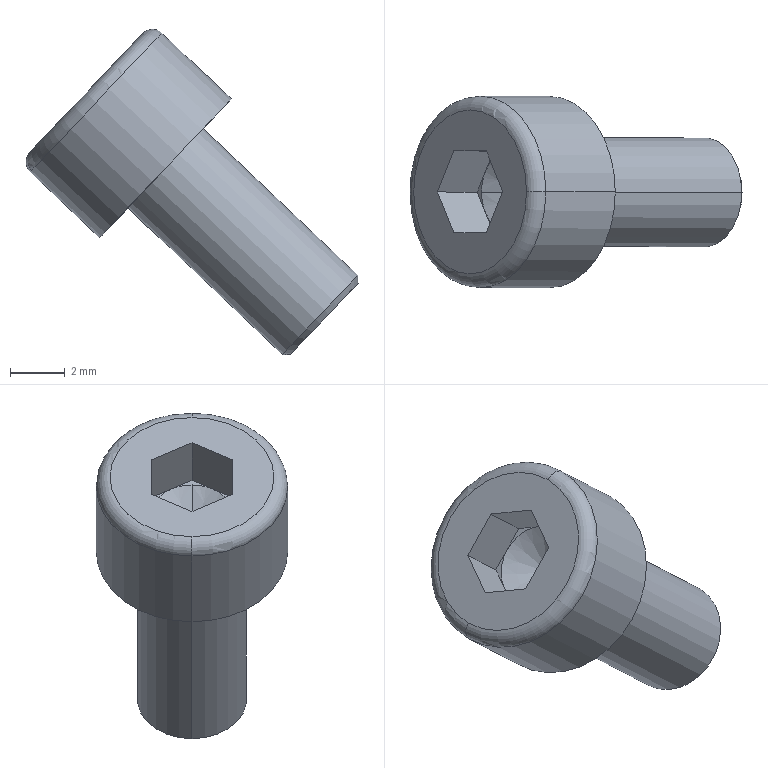Component | SolidWorks | 100-1_hexagon socket head cap screws gb_GB_FASTENER_SCREWS_HSHCS M4X8-N-1 | 1 solid | 25 faces | box 12.15 x 7 x 11.9 mm | volume 235 mm3 | plane 15 | cone 4 | cylinder 4 | torus 2 | commonest cylinder face diameters 4 x2 7 x2
STEP:
#1=COLOUR_RGB('',0.7922,0.8196,0.9333);
#2=FILL_AREA_STYLE_COLOUR('',#1);
#3=FILL_AREA_STYLE('',(#2));
#4=SURFACE_STYLE_FILL_AREA(#3);
#5=SURFACE_SIDE_STYLE('',(#4));
#6=SURFACE_STYLE_USAGE(.BOTH.,#5);
#7=PRESENTATION_STYLE_ASSIGNMENT((#6));
#8=CARTESIAN_POINT('',(20.34,50.315,-80.234));
#9=VERTEX_POINT('',#8);
#10=CARTESIAN_POINT('',(20.34,50.315,-80.222));
#11=VERTEX_POINT('',#10);
#12=CARTESIAN_POINT('',(20.34,50.315,-80.234));
#13=DIRECTION('',(-0.02683,-0.,0.9996));
#14=VECTOR('',#13,39.37);
#15=LINE('',#12,#14);
#16=EDGE_CURVE('',#9,#11,#15,.T.);
#17=ORIENTED_EDGE('',*,*,#16,.F.);
#18=CARTESIAN_POINT('',(20.242,50.315,-80.336));
#19=VERTEX_POINT('',#18);
#20=CARTESIAN_POINT('',(20.291,50.315,-80.285));
#21=DIRECTION('',(0.7258,0.,-0.6879));
#22=DIRECTION('',(0.6879,-0.,0.7258));
#23=AXIS2_PLACEMENT_3D('',#20,#21,#22);
#24=CIRCLE('',#23,0.07087);
#25=EDGE_CURVE('',#19,#9,#24,.T.);
#26=ORIENTED_EDGE('',*,*,#25,.F.);
#27=CARTESIAN_POINT('',(20.231,50.315,-80.337));
#28=VERTEX_POINT('',#27);
#29=CARTESIAN_POINT('',(20.242,50.315,-80.336));
#30=DIRECTION('',(-0.9996,0.,-0.02683));
#31=VECTOR('',#30,39.37);
#32=LINE('',#29,#31);
#33=EDGE_CURVE('',#19,#28,#32,.T.);
#34=ORIENTED_EDGE('',*,*,#33,.T.);
#35=CARTESIAN_POINT('',(20.285,50.315,-80.28));
#36=DIRECTION('',(-0.7258,-0.,0.6879));
#37=DIRECTION('',(0.6879,-0.,0.7258));
#38=AXIS2_PLACEMENT_3D('',#35,#36,#37);
#39=CIRCLE('',#38,0.07874);
#40=EDGE_CURVE('',#11,#28,#39,.T.);
#41=ORIENTED_EDGE('',*,*,#40,.F.);
#42=EDGE_LOOP('',(#17,#26,#34,#41));
#43=FACE_OUTER_BOUND('',#42,.T.);
#44=CARTESIAN_POINT('',(20.291,50.315,-80.285));
#45=DIRECTION('',(-0.7258,-0.,0.6879));
#46=DIRECTION('',(-0.6879,0.,-0.7258));
#47=AXIS2_PLACEMENT_3D('',#44,#45,#46);
#48=CONICAL_SURFACE('',#47,0.07087,0.7854);
#49=ADVANCED_FACE('',(#43),#48,.T.);
#50=CARTESIAN_POINT('',(19.867,50.315,-80.046));
#51=VERTEX_POINT('',#50);
#52=CARTESIAN_POINT('',(19.868,50.315,-80.074));
#53=VERTEX_POINT('',#52);
#54=CARTESIAN_POINT('',(19.881,50.315,-80.059));
#55=DIRECTION('',(-0.,-1.,-0.));
#56=DIRECTION('',(-0.6879,0.,-0.7258));
#57=AXIS2_PLACEMENT_3D('',#54,#55,#56);
#58=CIRCLE('',#57,0.01969);
#59=EDGE_CURVE('',#51,#53,#58,.T.);
#60=ORIENTED_EDGE('',*,*,#59,.F.);
#61=CARTESIAN_POINT('',(20.029,50.315,-79.874));
#62=VERTEX_POINT('',#61);
#63=CARTESIAN_POINT('',(19.948,50.315,-79.96));
#64=DIRECTION('',(-0.7258,-0.,0.6879));
#65=DIRECTION('',(0.6879,-0.,0.7258));
#66=AXIS2_PLACEMENT_3D('',#63,#64,#65);
#67=CIRCLE('',#66,0.1181);
#68=EDGE_CURVE('',#62,#51,#67,.T.);
#69=ORIENTED_EDGE('',*,*,#68,.F.);
#70=CARTESIAN_POINT('',(20.057,50.315,-79.874));
#71=VERTEX_POINT('',#70);
#72=CARTESIAN_POINT('',(20.044,50.315,-79.888));
#73=DIRECTION('',(0.,1.,0.));
#74=DIRECTION('',(0.6879,0.,0.7258));
#75=AXIS2_PLACEMENT_3D('',#72,#73,#74);
#76=CIRCLE('',#75,0.01969);
#77=EDGE_CURVE('',#62,#71,#76,.T.);
#78=ORIENTED_EDGE('',*,*,#77,.T.);
#79=CARTESIAN_POINT('',(19.963,50.315,-79.974));
#80=DIRECTION('',(0.7258,0.,-0.6879));
#81=DIRECTION('',(0.6879,-0.,0.7258));
#82=AXIS2_PLACEMENT_3D('',#79,#80,#81);
#83=CIRCLE('',#82,0.1378);
#84=EDGE_CURVE('',#53,#71,#83,.T.);
#85=ORIENTED_EDGE('',*,*,#84,.F.);
#86=EDGE_LOOP('',(#60,#69,#78,#85));
#87=FACE_OUTER_BOUND('',#86,.T.);
#88=CARTESIAN_POINT('',(19.963,50.315,-79.974));
#89=DIRECTION('',(0.7258,0.,-0.6879));
#90=DIRECTION('',(0.6879,-0.,0.7258));
#91=AXIS2_PLACEMENT_3D('',#88,#89,#90);
#92=TOROIDAL_SURFACE('',#91,0.1181,0.01969);
#93=ADVANCED_FACE('',(#87),#92,.T.);
#94=CARTESIAN_POINT('',(20.03,50.315,-80.038));
#95=VERTEX_POINT('',#94);
#96=CARTESIAN_POINT('',(20.046,50.315,-79.971));
#97=VERTEX_POINT('',#96);
#98=CARTESIAN_POINT('',(20.046,50.315,-79.971));
#99=DIRECTION('',(0.2328,-0.,0.9725));
#100=VECTOR('',#99,39.37);
#101=LINE('',#98,#100);
#102=EDGE_CURVE('',#95,#97,#101,.T.);
#103=ORIENTED_EDGE('',*,*,#102,.F.);
#104=CARTESIAN_POINT('',(19.965,50.315,-80.057));
#105=VERTEX_POINT('',#104);
#106=CARTESIAN_POINT('',(19.965,50.315,-80.057));
#107=DIRECTION('',(-0.9586,0.,-0.2846));
#108=VECTOR('',#107,39.37);
#109=LINE('',#106,#108);
#110=EDGE_CURVE('',#95,#105,#109,.T.);
#111=ORIENTED_EDGE('',*,*,#110,.T.);
#112=CARTESIAN_POINT('',(19.97,50.285,-80.051));
#113=VERTEX_POINT('',#112);
#114=CARTESIAN_POINT('',(20.005,50.315,-80.014));
#115=DIRECTION('',(-0.7258,-0.,0.6879));
#116=DIRECTION('',(0.6879,-0.,0.7258));
#117=AXIS2_PLACEMENT_3D('',#114,#115,#116);
#118=CIRCLE('',#117,0.05906);
#119=EDGE_CURVE('',#105,#113,#118,.T.);
#120=ORIENTED_EDGE('',*,*,#119,.T.);
#121=CARTESIAN_POINT('',(20.005,50.256,-80.014));
#122=VERTEX_POINT('',#121);
#123=CARTESIAN_POINT('',(20.005,50.315,-80.014));
#124=DIRECTION('',(-0.7258,-0.,0.6879));
#125=DIRECTION('',(0.6879,-0.,0.7258));
#126=AXIS2_PLACEMENT_3D('',#123,#124,#125);
#127=CIRCLE('',#126,0.05906);
#128=EDGE_CURVE('',#113,#122,#127,.T.);
#129=ORIENTED_EDGE('',*,*,#128,.T.);
#130=CARTESIAN_POINT('',(20.041,50.285,-79.977));
#131=VERTEX_POINT('',#130);
#132=CARTESIAN_POINT('',(20.005,50.315,-80.014));
#133=DIRECTION('',(0.7258,0.,-0.6879));
#134=DIRECTION('',(0.6879,-0.,0.7258));
#135=AXIS2_PLACEMENT_3D('',#132,#133,#134);
#136=CIRCLE('',#135,0.05906);
#137=EDGE_CURVE('',#131,#122,#136,.T.);
#138=ORIENTED_EDGE('',*,*,#137,.F.);
#139=CARTESIAN_POINT('',(20.005,50.315,-80.014));
#140=DIRECTION('',(-0.7258,-0.,0.6879));
#141=DIRECTION('',(0.6879,-0.,0.7258));
#142=AXIS2_PLACEMENT_3D('',#139,#140,#141);
#143=CIRCLE('',#142,0.05906);
#144=EDGE_CURVE('',#131,#97,#143,.T.);
#145=ORIENTED_EDGE('',*,*,#144,.T.);
#146=EDGE_LOOP('',(#103,#111,#120,#129,#138,#145));
#147=FACE_OUTER_BOUND('',#146,.T.);
#148=CARTESIAN_POINT('',(20.005,50.315,-80.014));
#149=DIRECTION('',(-0.7258,-0.,0.6879));
#150=DIRECTION('',(-0.6879,0.,-0.7258));
#151=AXIS2_PLACEMENT_3D('',#148,#149,#150);
#152=CONICAL_SURFACE('',#151,0.05906,1.047);
#153=ADVANCED_FACE('',(#147),#152,.F.);
#154=CARTESIAN_POINT('',(19.925,50.374,-79.985));
#155=VERTEX_POINT('',#154);
#156=CARTESIAN_POINT('',(19.972,50.374,-79.935));
#157=VERTEX_POINT('',#156);
#158=CARTESIAN_POINT('',(19.925,50.374,-79.985));
#159=DIRECTION('',(0.6879,-0.,0.7258));
#160=VECTOR('',#159,39.37);
#161=LINE('',#158,#160);
#162=EDGE_CURVE('',#155,#157,#161,.T.);
#163=ORIENTED_EDGE('',*,*,#162,.F.);
#164=CARTESIAN_POINT('',(19.982,50.374,-80.039));
#165=VERTEX_POINT('',#164);
#166=CARTESIAN_POINT('',(19.982,50.374,-80.039));
#167=DIRECTION('',(-0.7258,-0.,0.6879));
#168=VECTOR('',#167,39.37);
#169=LINE('',#166,#168);
#170=EDGE_CURVE('',#165,#155,#169,.T.);
#171=ORIENTED_EDGE('',*,*,#170,.F.);
#172=CARTESIAN_POINT('',(20.005,50.374,-80.014));
#173=VERTEX_POINT('',#172);
#174=CARTESIAN_POINT('',(19.982,50.374,-80.039));
#175=DIRECTION('',(0.6879,-0.,0.7258));
#176=VECTOR('',#175,39.37);
#177=LINE('',#174,#176);
#178=EDGE_CURVE('',#165,#173,#177,.T.);
#179=ORIENTED_EDGE('',*,*,#178,.T.);
#180=CARTESIAN_POINT('',(20.029,50.374,-79.989));
#181=VERTEX_POINT('',#180);
#182=CARTESIAN_POINT('',(19.982,50.374,-80.039));
#183=DIRECTION('',(0.6879,-0.,0.7258));
#184=VECTOR('',#183,39.37);
#185=LINE('',#182,#184);
#186=EDGE_CURVE('',#173,#181,#185,.T.);
#187=ORIENTED_EDGE('',*,*,#186,.T.);
#188=CARTESIAN_POINT('',(20.029,50.374,-79.989));
#189=DIRECTION('',(-0.7258,-0.,0.6879));
#190=VECTOR('',#189,39.37);
#191=LINE('',#188,#190);
#192=EDGE_CURVE('',#181,#157,#191,.T.);
#193=ORIENTED_EDGE('',*,*,#192,.T.);
#194=EDGE_LOOP('',(#163,#171,#179,#187,#193));
#195=FACE_OUTER_BOUND('',#194,.T.);
#196=CARTESIAN_POINT('',(19.982,50.374,-80.039));
#197=DIRECTION('',(-0.,-1.,-0.));
#198=DIRECTION('',(0.6879,-0.,0.7258));
#199=AXIS2_PLACEMENT_3D('',#196,#197,#198);
#200=PLANE('',#199);
#201=ADVANCED_FACE('',(#195),#200,.T.);
#202=CARTESIAN_POINT('',(19.901,50.315,-80.01));
#203=VERTEX_POINT('',#202);
#204=CARTESIAN_POINT('',(19.901,50.315,-80.01));
#205=DIRECTION('',(0.3439,0.866,0.3629));
#206=VECTOR('',#205,39.37);
#207=LINE('',#204,#206);
#208=EDGE_CURVE('',#203,#155,#207,.T.);
#209=ORIENTED_EDGE('',*,*,#208,.F.);
#210=CARTESIAN_POINT('',(19.958,50.315,-80.064));
#211=VERTEX_POINT('',#210);
#212=CARTESIAN_POINT('',(19.958,50.315,-80.064));
#213=DIRECTION('',(-0.7258,-0.,0.6879));
#214=VECTOR('',#213,39.37);
#215=LINE('',#212,#214);
#216=EDGE_CURVE('',#211,#203,#215,.T.);
#217=ORIENTED_EDGE('',*,*,#216,.F.);
#218=CARTESIAN_POINT('',(19.97,50.344,-80.051));
#219=VERTEX_POINT('',#218);
#220=CARTESIAN_POINT('',(19.958,50.315,-80.064));
#221=DIRECTION('',(0.3439,0.866,0.3629));
#222=VECTOR('',#221,39.37);
#223=LINE('',#220,#222);
#224=EDGE_CURVE('',#211,#219,#223,.T.);
#225=ORIENTED_EDGE('',*,*,#224,.T.);
#226=CARTESIAN_POINT('',(19.958,50.315,-80.064));
#227=DIRECTION('',(0.3439,0.866,0.3629));
#228=VECTOR('',#227,39.37);
#229=LINE('',#226,#228);
#230=EDGE_CURVE('',#219,#165,#229,.T.);
#231=ORIENTED_EDGE('',*,*,#230,.T.);
#232=ORIENTED_EDGE('',*,*,#170,.T.);
#233=EDGE_LOOP('',(#209,#217,#225,#231,#232));
#234=FACE_OUTER_BOUND('',#233,.T.);
#235=CARTESIAN_POINT('',(19.958,50.315,-80.064));
#236=DIRECTION('',(0.5957,-0.5,0.6286));
#237=DIRECTION('',(-0.7258,-0.,0.6879));
#238=AXIS2_PLACEMENT_3D('',#235,#236,#237);
#239=PLANE('',#238);
#240=ADVANCED_FACE('',(#234),#239,.T.);
#241=CARTESIAN_POINT('',(19.925,50.256,-79.985));
#242=VERTEX_POINT('',#241);
#243=CARTESIAN_POINT('',(19.925,50.256,-79.985));
#244=DIRECTION('',(-0.3439,0.866,-0.3629));
#245=VECTOR('',#244,39.37);
#246=LINE('',#243,#245);
#247=EDGE_CURVE('',#242,#203,#246,.T.);
#248=ORIENTED_EDGE('',*,*,#247,.F.);
#249=CARTESIAN_POINT('',(19.982,50.256,-80.039));
#250=VERTEX_POINT('',#249);
#251=CARTESIAN_POINT('',(19.982,50.256,-80.039));
#252=DIRECTION('',(-0.7258,-0.,0.6879));
#253=VECTOR('',#252,39.37);
#254=LINE('',#251,#253);
#255=EDGE_CURVE('',#250,#242,#254,.T.);
#256=ORIENTED_EDGE('',*,*,#255,.F.);
#257=CARTESIAN_POINT('',(19.982,50.256,-80.039));
#258=DIRECTION('',(-0.3439,0.866,-0.3629));
#259=VECTOR('',#258,39.37);
#260=LINE('',#257,#259);
#261=EDGE_CURVE('',#250,#113,#260,.T.);
#262=ORIENTED_EDGE('',*,*,#261,.T.);
#263=CARTESIAN_POINT('',(19.982,50.256,-80.039));
#264=DIRECTION('',(-0.3439,0.866,-0.3629));
#265=VECTOR('',#264,39.37);
#266=LINE('',#263,#265);
#267=EDGE_CURVE('',#113,#211,#266,.T.);
#268=ORIENTED_EDGE('',*,*,#267,.T.);
#269=ORIENTED_EDGE('',*,*,#216,.T.);
#270=EDGE_LOOP('',(#248,#256,#262,#268,#269));
#271=FACE_OUTER_BOUND('',#270,.T.);
#272=CARTESIAN_POINT('',(19.982,50.256,-80.039));
#273=DIRECTION('',(0.5957,0.5,0.6286));
#274=DIRECTION('',(-0.3439,0.866,-0.3629));
#275=AXIS2_PLACEMENT_3D('',#272,#273,#274);
#276=PLANE('',#275);
#277=ADVANCED_FACE('',(#271),#276,.T.);
#278=CARTESIAN_POINT('',(19.972,50.256,-79.935));
#279=VERTEX_POINT('',#278);
#280=CARTESIAN_POINT('',(19.972,50.256,-79.935));
#281=DIRECTION('',(-0.6879,0.,-0.7258));
#282=VECTOR('',#281,39.37);
#283=LINE('',#280,#282);
#284=EDGE_CURVE('',#279,#242,#283,.T.);
#285=ORIENTED_EDGE('',*,*,#284,.F.);
#286=CARTESIAN_POINT('',(20.029,50.256,-79.989));
#287=VERTEX_POINT('',#286);
#288=CARTESIAN_POINT('',(20.029,50.256,-79.989));
#289=DIRECTION('',(-0.7258,-0.,0.6879));
#290=VECTOR('',#289,39.37);
#291=LINE('',#288,#290);
#292=EDGE_CURVE('',#287,#279,#291,.T.);
#293=ORIENTED_EDGE('',*,*,#292,.F.);
#294=CARTESIAN_POINT('',(20.029,50.256,-79.989));
#295=DIRECTION('',(-0.6879,0.,-0.7258));
#296=VECTOR('',#295,39.37);
#297=LINE('',#294,#296);
#298=EDGE_CURVE('',#287,#122,#297,.T.);
#299=ORIENTED_EDGE('',*,*,#298,.T.);
#300=CARTESIAN_POINT('',(20.029,50.256,-79.989));
#301=DIRECTION('',(-0.6879,0.,-0.7258));
#302=VECTOR('',#301,39.37);
#303=LINE('',#300,#302);
#304=EDGE_CURVE('',#122,#250,#303,.T.);
#305=ORIENTED_EDGE('',*,*,#304,.T.);
#306=ORIENTED_EDGE('',*,*,#255,.T.);
#307=EDGE_LOOP('',(#285,#293,#299,#305,#306));
#308=FACE_OUTER_BOUND('',#307,.T.);
#309=CARTESIAN_POINT('',(20.029,50.256,-79.989));
#310=DIRECTION('',(0.,1.,0.));
#311=DIRECTION('',(0.6879,-0.,0.7258));
#312=AXIS2_PLACEMENT_3D('',#309,#310,#311);
#313=PLANE('',#312);
#314=ADVANCED_FACE('',(#308),#313,.T.);
#315=CARTESIAN_POINT('',(19.995,50.315,-79.911));
#316=VERTEX_POINT('',#315);
#317=CARTESIAN_POINT('',(19.995,50.315,-79.911));
#318=DIRECTION('',(-0.3439,-0.866,-0.3629));
#319=VECTOR('',#318,39.37);
#320=LINE('',#317,#319);
#321=EDGE_CURVE('',#316,#279,#320,.T.);
#322=ORIENTED_EDGE('',*,*,#321,.F.);
#323=CARTESIAN_POINT('',(20.052,50.315,-79.965));
#324=VERTEX_POINT('',#323);
#325=CARTESIAN_POINT('',(20.052,50.315,-79.965));
#326=DIRECTION('',(-0.7258,-0.,0.6879));
#327=VECTOR('',#326,39.37);
#328=LINE('',#325,#327);
#329=EDGE_CURVE('',#324,#316,#328,.T.);
#330=ORIENTED_EDGE('',*,*,#329,.F.);
#331=CARTESIAN_POINT('',(20.052,50.315,-79.965));
#332=DIRECTION('',(-0.3439,-0.866,-0.3629));
#333=VECTOR('',#332,39.37);
#334=LINE('',#331,#333);
#335=EDGE_CURVE('',#324,#131,#334,.T.);
#336=ORIENTED_EDGE('',*,*,#335,.T.);
#337=CARTESIAN_POINT('',(20.052,50.315,-79.965));
#338=DIRECTION('',(-0.3439,-0.866,-0.3629));
#339=VECTOR('',#338,39.37);
#340=LINE('',#337,#339);
#341=EDGE_CURVE('',#131,#287,#340,.T.);
#342=ORIENTED_EDGE('',*,*,#341,.T.);
#343=ORIENTED_EDGE('',*,*,#292,.T.);
#344=EDGE_LOOP('',(#322,#330,#336,#342,#343));
#345=FACE_OUTER_BOUND('',#344,.T.);
#346=CARTESIAN_POINT('',(20.052,50.315,-79.965));
#347=DIRECTION('',(-0.5957,0.5,-0.6286));
#348=DIRECTION('',(-0.7258,-0.,0.6879));
#349=AXIS2_PLACEMENT_3D('',#346,#347,#348);
#350=PLANE('',#349);
#351=ADVANCED_FACE('',(#345),#350,.T.);
#352=CARTESIAN_POINT('',(19.972,50.374,-79.935));
#353=DIRECTION('',(0.3439,-0.866,0.3629));
#354=VECTOR('',#353,39.37);
#355=LINE('',#352,#354);
#356=EDGE_CURVE('',#157,#316,#355,.T.);
#357=ORIENTED_EDGE('',*,*,#356,.F.);
#358=ORIENTED_EDGE('',*,*,#192,.F.);
#359=CARTESIAN_POINT('',(20.041,50.344,-79.977));
#360=VERTEX_POINT('',#359);
#361=CARTESIAN_POINT('',(20.029,50.374,-79.989));
#362=DIRECTION('',(0.3439,-0.866,0.3629));
#363=VECTOR('',#362,39.37);
#364=LINE('',#361,#363);
#365=EDGE_CURVE('',#181,#360,#364,.T.);
#366=ORIENTED_EDGE('',*,*,#365,.T.);
#367=CARTESIAN_POINT('',(20.029,50.374,-79.989));
#368=DIRECTION('',(0.3439,-0.866,0.3629));
#369=VECTOR('',#368,39.37);
#370=LINE('',#367,#369);
#371=EDGE_CURVE('',#360,#324,#370,.T.);
#372=ORIENTED_EDGE('',*,*,#371,.T.);
#373=ORIENTED_EDGE('',*,*,#329,.T.);
#374=EDGE_LOOP('',(#357,#358,#366,#372,#373));
#375=FACE_OUTER_BOUND('',#374,.T.);
#376=CARTESIAN_POINT('',(20.029,50.374,-79.989));
#377=DIRECTION('',(-0.5957,-0.5,-0.6286));
#378=DIRECTION('',(0.7258,0.,-0.6879));
#379=AXIS2_PLACEMENT_3D('',#376,#377,#378);
#380=PLANE('',#379);
#381=ADVANCED_FACE('',(#375),#380,.T.);
#382=ORIENTED_EDGE('',*,*,#25,.T.);
#383=CARTESIAN_POINT('',(20.291,50.315,-80.285));
#384=DIRECTION('',(0.7258,0.,-0.6879));
#385=DIRECTION('',(0.6879,-0.,0.7258));
#386=AXIS2_PLACEMENT_3D('',#383,#384,#385);
#387=CIRCLE('',#386,0.07087);
#388=EDGE_CURVE('',#9,#19,#387,.T.);
#389=ORIENTED_EDGE('',*,*,#388,.T.);
#390=EDGE_LOOP('',(#382,#389));
#391=FACE_OUTER_BOUND('',#390,.T.);
#392=CARTESIAN_POINT('',(20.291,50.315,-80.285));
#393=DIRECTION('',(0.7258,0.,-0.6879));
#394=DIRECTION('',(-0.,-1.,-0.));
#395=AXIS2_PLACEMENT_3D('',#392,#393,#394);
#396=PLANE('',#395);
#397=ADVANCED_FACE('',(#391),#396,.T.);
#398=CARTESIAN_POINT('',(20.117,50.315,-80.011));
#399=VERTEX_POINT('',#398);
#400=CARTESIAN_POINT('',(20.345,50.315,-80.228));
#401=DIRECTION('',(-0.7258,-0.,0.6879));
#402=VECTOR('',#401,39.37);
#403=LINE('',#400,#402);
#404=EDGE_CURVE('',#11,#399,#403,.T.);
#405=ORIENTED_EDGE('',*,*,#404,.F.);
#406=ORIENTED_EDGE('',*,*,#40,.T.);
#407=CARTESIAN_POINT('',(20.008,50.315,-80.126));
#408=VERTEX_POINT('',#407);
#409=CARTESIAN_POINT('',(20.237,50.315,-80.342));
#410=DIRECTION('',(-0.7258,-0.,0.6879));
#411=VECTOR('',#410,39.37);
#412=LINE('',#409,#411);
#413=EDGE_CURVE('',#28,#408,#412,.T.);
#414=ORIENTED_EDGE('',*,*,#413,.T.);
#415=CARTESIAN_POINT('',(20.063,50.315,-80.068));
#416=DIRECTION('',(0.7258,0.,-0.6879));
#417=DIRECTION('',(0.6879,-0.,0.7258));
#418=AXIS2_PLACEMENT_3D('',#415,#416,#417);
#419=CIRCLE('',#418,0.07874);
#420=EDGE_CURVE('',#408,#399,#419,.T.);
#421=ORIENTED_EDGE('',*,*,#420,.T.);
#422=EDGE_LOOP('',(#405,#406,#414,#421));
#423=FACE_OUTER_BOUND('',#422,.T.);
#424=CARTESIAN_POINT('',(20.291,50.315,-80.285));
#425=DIRECTION('',(-0.7258,-0.,0.6879));
#426=DIRECTION('',(-0.6879,0.,-0.7258));
#427=AXIS2_PLACEMENT_3D('',#424,#425,#426);
#428=CYLINDRICAL_SURFACE('',#427,0.07874);
#429=ADVANCED_FACE('',(#423),#428,.T.);
#430=CARTESIAN_POINT('',(20.157,50.315,-79.968));
#431=VERTEX_POINT('',#430);
#432=CARTESIAN_POINT('',(20.157,50.315,-79.968));
#433=DIRECTION('',(-0.7258,-0.,0.6879));
#434=VECTOR('',#433,39.37);
#435=LINE('',#432,#434);
#436=EDGE_CURVE('',#431,#71,#435,.T.);
#437=ORIENTED_EDGE('',*,*,#436,.F.);
#438=CARTESIAN_POINT('',(19.968,50.315,-80.168));
#439=VERTEX_POINT('',#438);
#440=CARTESIAN_POINT('',(20.063,50.315,-80.068));
#441=DIRECTION('',(0.7258,0.,-0.6879));
#442=DIRECTION('',(0.6879,-0.,0.7258));
#443=AXIS2_PLACEMENT_3D('',#440,#441,#442);
#444=CIRCLE('',#443,0.1378);
#445=EDGE_CURVE('',#439,#431,#444,.T.);
#446=ORIENTED_EDGE('',*,*,#445,.F.);
#447=CARTESIAN_POINT('',(19.968,50.315,-80.168));
#448=DIRECTION('',(-0.7258,-0.,0.6879));
#449=VECTOR('',#448,39.37);
#450=LINE('',#447,#449);
#451=EDGE_CURVE('',#439,#53,#450,.T.);
#452=ORIENTED_EDGE('',*,*,#451,.T.);
#453=ORIENTED_EDGE('',*,*,#84,.T.);
#454=EDGE_LOOP('',(#437,#446,#452,#453));
#455=FACE_OUTER_BOUND('',#454,.T.);
#456=CARTESIAN_POINT('',(20.063,50.315,-80.068));
#457=DIRECTION('',(-0.7258,-0.,0.6879));
#458=DIRECTION('',(-0.6879,0.,-0.7258));
#459=AXIS2_PLACEMENT_3D('',#456,#457,#458);
#460=CYLINDRICAL_SURFACE('',#459,0.1378);
#461=ADVANCED_FACE('',(#455),#460,.T.);
#462=ORIENTED_EDGE('',*,*,#420,.F.);
#463=CARTESIAN_POINT('',(20.063,50.315,-80.068));
#464=DIRECTION('',(0.7258,0.,-0.6879));
#465=DIRECTION('',(0.6879,-0.,0.7258));
#466=AXIS2_PLACEMENT_3D('',#463,#464,#465);
#467=CIRCLE('',#466,0.07874);
#468=EDGE_CURVE('',#399,#408,#467,.T.);
#469=ORIENTED_EDGE('',*,*,#468,.F.);
#470=EDGE_LOOP('',(#462,#469));
#471=FACE_BOUND('',#470,.T.);
#472=ORIENTED_EDGE('',*,*,#445,.T.);
#473=CARTESIAN_POINT('',(20.063,50.315,-80.068));
#474=DIRECTION('',(0.7258,0.,-0.6879));
#475=DIRECTION('',(0.6879,-0.,0.7258));
#476=AXIS2_PLACEMENT_3D('',#473,#474,#475);
#477=CIRCLE('',#476,0.1378);
#478=EDGE_CURVE('',#431,#439,#477,.T.);
#479=ORIENTED_EDGE('',*,*,#478,.T.);
#480=EDGE_LOOP('',(#472,#479));
#481=FACE_OUTER_BOUND('',#480,.T.);
#482=CARTESIAN_POINT('',(20.063,50.315,-80.068));
#483=DIRECTION('',(0.7258,0.,-0.6879));
#484=DIRECTION('',(-0.,-1.,-0.));
#485=AXIS2_PLACEMENT_3D('',#482,#483,#484);
#486=PLANE('',#485);
#487=ADVANCED_FACE('',(#471,#481),#486,.T.);
#488=ORIENTED_EDGE('',*,*,#356,.T.);
#489=ORIENTED_EDGE('',*,*,#321,.T.);
#490=ORIENTED_EDGE('',*,*,#284,.T.);
#491=ORIENTED_EDGE('',*,*,#247,.T.);
#492=ORIENTED_EDGE('',*,*,#208,.T.);
#493=ORIENTED_EDGE('',*,*,#162,.T.);
#494=EDGE_LOOP('',(#488,#489,#490,#491,#492,#493));
#495=FACE_BOUND('',#494,.T.);
#496=ORIENTED_EDGE('',*,*,#68,.T.);
#497=CARTESIAN_POINT('',(19.948,50.315,-79.96));
#498=DIRECTION('',(-0.7258,-0.,0.6879));
#499=DIRECTION('',(0.6879,-0.,0.7258));
#500=AXIS2_PLACEMENT_3D('',#497,#498,#499);
#501=CIRCLE('',#500,0.1181);
#502=EDGE_CURVE('',#51,#62,#501,.T.);
#503=ORIENTED_EDGE('',*,*,#502,.T.);
#504=EDGE_LOOP('',(#496,#503));
#505=FACE_OUTER_BOUND('',#504,.T.);
#506=CARTESIAN_POINT('',(19.948,50.315,-79.96));
#507=DIRECTION('',(0.7258,0.,-0.6879));
#508=DIRECTION('',(-0.,-1.,-0.));
#509=AXIS2_PLACEMENT_3D('',#506,#507,#508);
#510=PLANE('',#509);
#511=ADVANCED_FACE('',(#495,#505),#510,.F.);
#512=ORIENTED_EDGE('',*,*,#144,.F.);
#513=ORIENTED_EDGE('',*,*,#335,.F.);
#514=ORIENTED_EDGE('',*,*,#371,.F.);
#515=CARTESIAN_POINT('',(20.005,50.315,-80.014));
#516=DIRECTION('',(-0.7258,-0.,0.6879));
#517=DIRECTION('',(0.6879,-0.,0.7258));
#518=AXIS2_PLACEMENT_3D('',#515,#516,#517);
#519=CIRCLE('',#518,0.05906);
#520=EDGE_CURVE('',#97,#360,#519,.T.);
#521=ORIENTED_EDGE('',*,*,#520,.F.);
#522=EDGE_LOOP('',(#512,#513,#514,#521));
#523=FACE_OUTER_BOUND('',#522,.T.);
#524=CARTESIAN_POINT('',(20.052,50.315,-79.965));
#525=DIRECTION('',(0.7258,0.,-0.6879));
#526=DIRECTION('',(-0.,-1.,-0.));
#527=AXIS2_PLACEMENT_3D('',#524,#525,#526);
#528=PLANE('',#527);
#529=ADVANCED_FACE('',(#523),#528,.F.);
#530=ORIENTED_EDGE('',*,*,#137,.T.);
#531=ORIENTED_EDGE('',*,*,#298,.F.);
#532=ORIENTED_EDGE('',*,*,#341,.F.);
#533=EDGE_LOOP('',(#530,#531,#532));
#534=FACE_OUTER_BOUND('',#533,.T.);
#535=CARTESIAN_POINT('',(20.052,50.315,-79.965));
#536=DIRECTION('',(0.7258,0.,-0.6879));
#537=DIRECTION('',(-0.,-1.,-0.));
#538=AXIS2_PLACEMENT_3D('',#535,#536,#537);
#539=PLANE('',#538);
#540=ADVANCED_FACE('',(#534),#539,.F.);
#541=ORIENTED_EDGE('',*,*,#128,.F.);
#542=ORIENTED_EDGE('',*,*,#261,.F.);
#543=ORIENTED_EDGE('',*,*,#304,.F.);
#544=EDGE_LOOP('',(#541,#542,#543));
#545=FACE_OUTER_BOUND('',#544,.T.);
#546=CARTESIAN_POINT('',(20.052,50.315,-79.965));
#547=DIRECTION('',(0.7258,0.,-0.6879));
#548=DIRECTION('',(-0.,-1.,-0.));
#549=AXIS2_PLACEMENT_3D('',#546,#547,#548);
#550=PLANE('',#549);
#551=ADVANCED_FACE('',(#545),#550,.F.);
#552=CARTESIAN_POINT('',(20.005,50.315,-80.014));
#553=DIRECTION('',(-0.7258,-0.,0.6879));
#554=DIRECTION('',(0.6879,-0.,0.7258));
#555=AXIS2_PLACEMENT_3D('',#552,#553,#554);
#556=CIRCLE('',#555,0.05906);
#557=EDGE_CURVE('',#219,#105,#556,.T.);
#558=ORIENTED_EDGE('',*,*,#557,.F.);
#559=ORIENTED_EDGE('',*,*,#224,.F.);
#560=ORIENTED_EDGE('',*,*,#267,.F.);
#561=ORIENTED_EDGE('',*,*,#119,.F.);
#562=EDGE_LOOP('',(#558,#559,#560,#561));
#563=FACE_OUTER_BOUND('',#562,.T.);
#564=CARTESIAN_POINT('',(20.052,50.315,-79.965));
#565=DIRECTION('',(0.7258,0.,-0.6879));
#566=DIRECTION('',(-0.,-1.,-0.));
#567=AXIS2_PLACEMENT_3D('',#564,#565,#566);
#568=PLANE('',#567);
#569=ADVANCED_FACE('',(#563),#568,.F.);
#570=CARTESIAN_POINT('',(20.005,50.315,-80.014));
#571=DIRECTION('',(-0.7258,-0.,0.6879));
#572=DIRECTION('',(0.6879,-0.,0.7258));
#573=AXIS2_PLACEMENT_3D('',#570,#571,#572);
#574=CIRCLE('',#573,0.05906);
#575=EDGE_CURVE('',#173,#219,#574,.T.);
#576=ORIENTED_EDGE('',*,*,#575,.F.);
#577=ORIENTED_EDGE('',*,*,#178,.F.);
#578=ORIENTED_EDGE('',*,*,#230,.F.);
#579=EDGE_LOOP('',(#576,#577,#578));
#580=FACE_OUTER_BOUND('',#579,.T.);
#581=CARTESIAN_POINT('',(20.052,50.315,-79.965));
#582=DIRECTION('',(0.7258,0.,-0.6879));
#583=DIRECTION('',(-0.,-1.,-0.));
#584=AXIS2_PLACEMENT_3D('',#581,#582,#583);
#585=PLANE('',#584);
#586=ADVANCED_FACE('',(#580),#585,.F.);
#587=CARTESIAN_POINT('',(20.005,50.315,-80.014));
#588=DIRECTION('',(-0.7258,-0.,0.6879));
#589=DIRECTION('',(0.6879,-0.,0.7258));
#590=AXIS2_PLACEMENT_3D('',#587,#588,#589);
#591=CIRCLE('',#590,0.05906);
#592=EDGE_CURVE('',#360,#173,#591,.T.);
#593=ORIENTED_EDGE('',*,*,#592,.F.);
#594=ORIENTED_EDGE('',*,*,#365,.F.);
#595=ORIENTED_EDGE('',*,*,#186,.F.);
#596=EDGE_LOOP('',(#593,#594,#595));
#597=FACE_OUTER_BOUND('',#596,.T.);
#598=CARTESIAN_POINT('',(20.052,50.315,-79.965));
#599=DIRECTION('',(0.7258,0.,-0.6879));
#600=DIRECTION('',(-0.,-1.,-0.));
#601=AXIS2_PLACEMENT_3D('',#598,#599,#600);
#602=PLANE('',#601);
#603=ADVANCED_FACE('',(#597),#602,.F.);
#604=ORIENTED_EDGE('',*,*,#478,.F.);
#605=ORIENTED_EDGE('',*,*,#436,.T.);
#606=CARTESIAN_POINT('',(19.963,50.315,-79.974));
#607=DIRECTION('',(0.7258,0.,-0.6879));
#608=DIRECTION('',(0.6879,-0.,0.7258));
#609=AXIS2_PLACEMENT_3D('',#606,#607,#608);
#610=CIRCLE('',#609,0.1378);
#611=EDGE_CURVE('',#71,#53,#610,.T.);
#612=ORIENTED_EDGE('',*,*,#611,.T.);
#613=ORIENTED_EDGE('',*,*,#451,.F.);
#614=EDGE_LOOP('',(#604,#605,#612,#613));
#615=FACE_OUTER_BOUND('',#614,.T.);
#616=CARTESIAN_POINT('',(20.063,50.315,-80.068));
#617=DIRECTION('',(-0.7258,-0.,0.6879));
#618=DIRECTION('',(-0.6879,0.,-0.7258));
#619=AXIS2_PLACEMENT_3D('',#616,#617,#618);
#620=CYLINDRICAL_SURFACE('',#619,0.1378);
#621=ADVANCED_FACE('',(#615),#620,.T.);
#622=CARTESIAN_POINT('',(20.285,50.315,-80.28));
#623=DIRECTION('',(-0.7258,-0.,0.6879));
#624=DIRECTION('',(0.6879,-0.,0.7258));
#625=AXIS2_PLACEMENT_3D('',#622,#623,#624);
#626=CIRCLE('',#625,0.07874);
#627=EDGE_CURVE('',#28,#11,#626,.T.);
#628=ORIENTED_EDGE('',*,*,#627,.T.);
#629=ORIENTED_EDGE('',*,*,#404,.T.);
#630=ORIENTED_EDGE('',*,*,#468,.T.);
#631=ORIENTED_EDGE('',*,*,#413,.F.);
#632=EDGE_LOOP('',(#628,#629,#630,#631));
#633=FACE_OUTER_BOUND('',#632,.T.);
#634=CARTESIAN_POINT('',(20.291,50.315,-80.285));
#635=DIRECTION('',(-0.7258,-0.,0.6879));
#636=DIRECTION('',(-0.6879,0.,-0.7258));
#637=AXIS2_PLACEMENT_3D('',#634,#635,#636);
#638=CYLINDRICAL_SURFACE('',#637,0.07874);
#639=ADVANCED_FACE('',(#633),#638,.T.);
#640=ORIENTED_EDGE('',*,*,#110,.F.);
#641=ORIENTED_EDGE('',*,*,#102,.T.);
#642=ORIENTED_EDGE('',*,*,#520,.T.);
#643=ORIENTED_EDGE('',*,*,#592,.T.);
#644=ORIENTED_EDGE('',*,*,#575,.T.);
#645=ORIENTED_EDGE('',*,*,#557,.T.);
#646=EDGE_LOOP('',(#640,#641,#642,#643,#644,#645));
#647=FACE_OUTER_BOUND('',#646,.T.);
#648=CARTESIAN_POINT('',(20.005,50.315,-80.014));
#649=DIRECTION('',(-0.7258,-0.,0.6879));
#650=DIRECTION('',(-0.6879,0.,-0.7258));
#651=AXIS2_PLACEMENT_3D('',#648,#649,#650);
#652=CONICAL_SURFACE('',#651,0.05906,1.047);
#653=ADVANCED_FACE('',(#647),#652,.F.);
#654=ORIENTED_EDGE('',*,*,#502,.F.);
#655=ORIENTED_EDGE('',*,*,#59,.T.);
#656=ORIENTED_EDGE('',*,*,#611,.F.);
#657=ORIENTED_EDGE('',*,*,#77,.F.);
#658=EDGE_LOOP('',(#654,#655,#656,#657));
#659=FACE_OUTER_BOUND('',#658,.T.);
#660=CARTESIAN_POINT('',(19.963,50.315,-79.974));
#661=DIRECTION('',(0.7258,0.,-0.6879));
#662=DIRECTION('',(0.6879,-0.,0.7258));
#663=AXIS2_PLACEMENT_3D('',#660,#661,#662);
#664=TOROIDAL_SURFACE('',#663,0.1181,0.01969);
#665=ADVANCED_FACE('',(#659),#664,.T.);
#666=ORIENTED_EDGE('',*,*,#388,.F.);
#667=ORIENTED_EDGE('',*,*,#16,.T.);
#668=ORIENTED_EDGE('',*,*,#627,.F.);
#669=ORIENTED_EDGE('',*,*,#33,.F.);
#670=EDGE_LOOP('',(#666,#667,#668,#669));
#671=FACE_OUTER_BOUND('',#670,.T.);
#672=CARTESIAN_POINT('',(20.291,50.315,-80.285));
#673=DIRECTION('',(-0.7258,-0.,0.6879));
#674=DIRECTION('',(-0.6879,0.,-0.7258));
#675=AXIS2_PLACEMENT_3D('',#672,#673,#674);
#676=CONICAL_SURFACE('',#675,0.07087,0.7854);
#677=ADVANCED_FACE('',(#671),#676,.T.);
#678=CLOSED_SHELL('',(#49,#93,#153,#201,#240,#277,#314,#351,#381,#397,#429,#461,#487,#511,#529,#540,#551,#569,#586,#603,#621,#639,#653,#665,#677));
#679=MANIFOLD_SOLID_BREP('',#678);
#680=STYLED_ITEM('',(#7),#679);
#681=PRESENTATION_LAYER_ASSIGNMENT('','',(#680));
#682=CARTESIAN_POINT('',(0.,0.,0.));
#683=DIRECTION('',(0.,0.,1.));
#684=DIRECTION('',(1.,0.,0.));
#685=AXIS2_PLACEMENT_3D('',#682,#683,#684);
#686=(LENGTH_UNIT()NAMED_UNIT(*)SI_UNIT($,.METRE.));
#687=LENGTH_MEASURE_WITH_UNIT(LENGTH_MEASURE(0.0254),#686);
#688=DIMENSIONAL_EXPONENTS(1.,0.,0.,0.,0.,0.,0.);
#689=(CONVERSION_BASED_UNIT('',#687)LENGTH_UNIT()NAMED_UNIT(#688));
#690=UNCERTAINTY_MEASURE_WITH_UNIT(LENGTH_MEASURE(0.00001),#689,'','');
#691=(NAMED_UNIT(*)PLANE_ANGLE_UNIT()SI_UNIT($,.RADIAN.));
#692=(NAMED_UNIT(*)SI_UNIT($,.STERADIAN.)SOLID_ANGLE_UNIT());
#693=(GEOMETRIC_REPRESENTATION_CONTEXT(3)GLOBAL_UNCERTAINTY_ASSIGNED_CONTEXT((#690))GLOBAL_UNIT_ASSIGNED_CONTEXT((#689,#691,#692))REPRESENTATION_CONTEXT('',''));
#694=ADVANCED_BREP_SHAPE_REPRESENTATION('',(#679,#685),#693);
#695=(LENGTH_UNIT()NAMED_UNIT(*)SI_UNIT($,.METRE.));
#696=LENGTH_MEASURE_WITH_UNIT(LENGTH_MEASURE(0.0254),#695);
#697=DIMENSIONAL_EXPONENTS(1.,0.,0.,0.,0.,0.,0.);
#698=(CONVERSION_BASED_UNIT('',#696)LENGTH_UNIT()NAMED_UNIT(#697));
#699=UNCERTAINTY_MEASURE_WITH_UNIT(LENGTH_MEASURE(0.00001),#698,'','');
#700=(NAMED_UNIT(*)PLANE_ANGLE_UNIT()SI_UNIT($,.RADIAN.));
#701=(NAMED_UNIT(*)SI_UNIT($,.STERADIAN.)SOLID_ANGLE_UNIT());
#702=(GEOMETRIC_REPRESENTATION_CONTEXT(3)GLOBAL_UNCERTAINTY_ASSIGNED_CONTEXT((#699))GLOBAL_UNIT_ASSIGNED_CONTEXT((#698,#700,#701))REPRESENTATION_CONTEXT('',''));
#703=MECHANICAL_DESIGN_GEOMETRIC_PRESENTATION_REPRESENTATION('',(#680),#702);